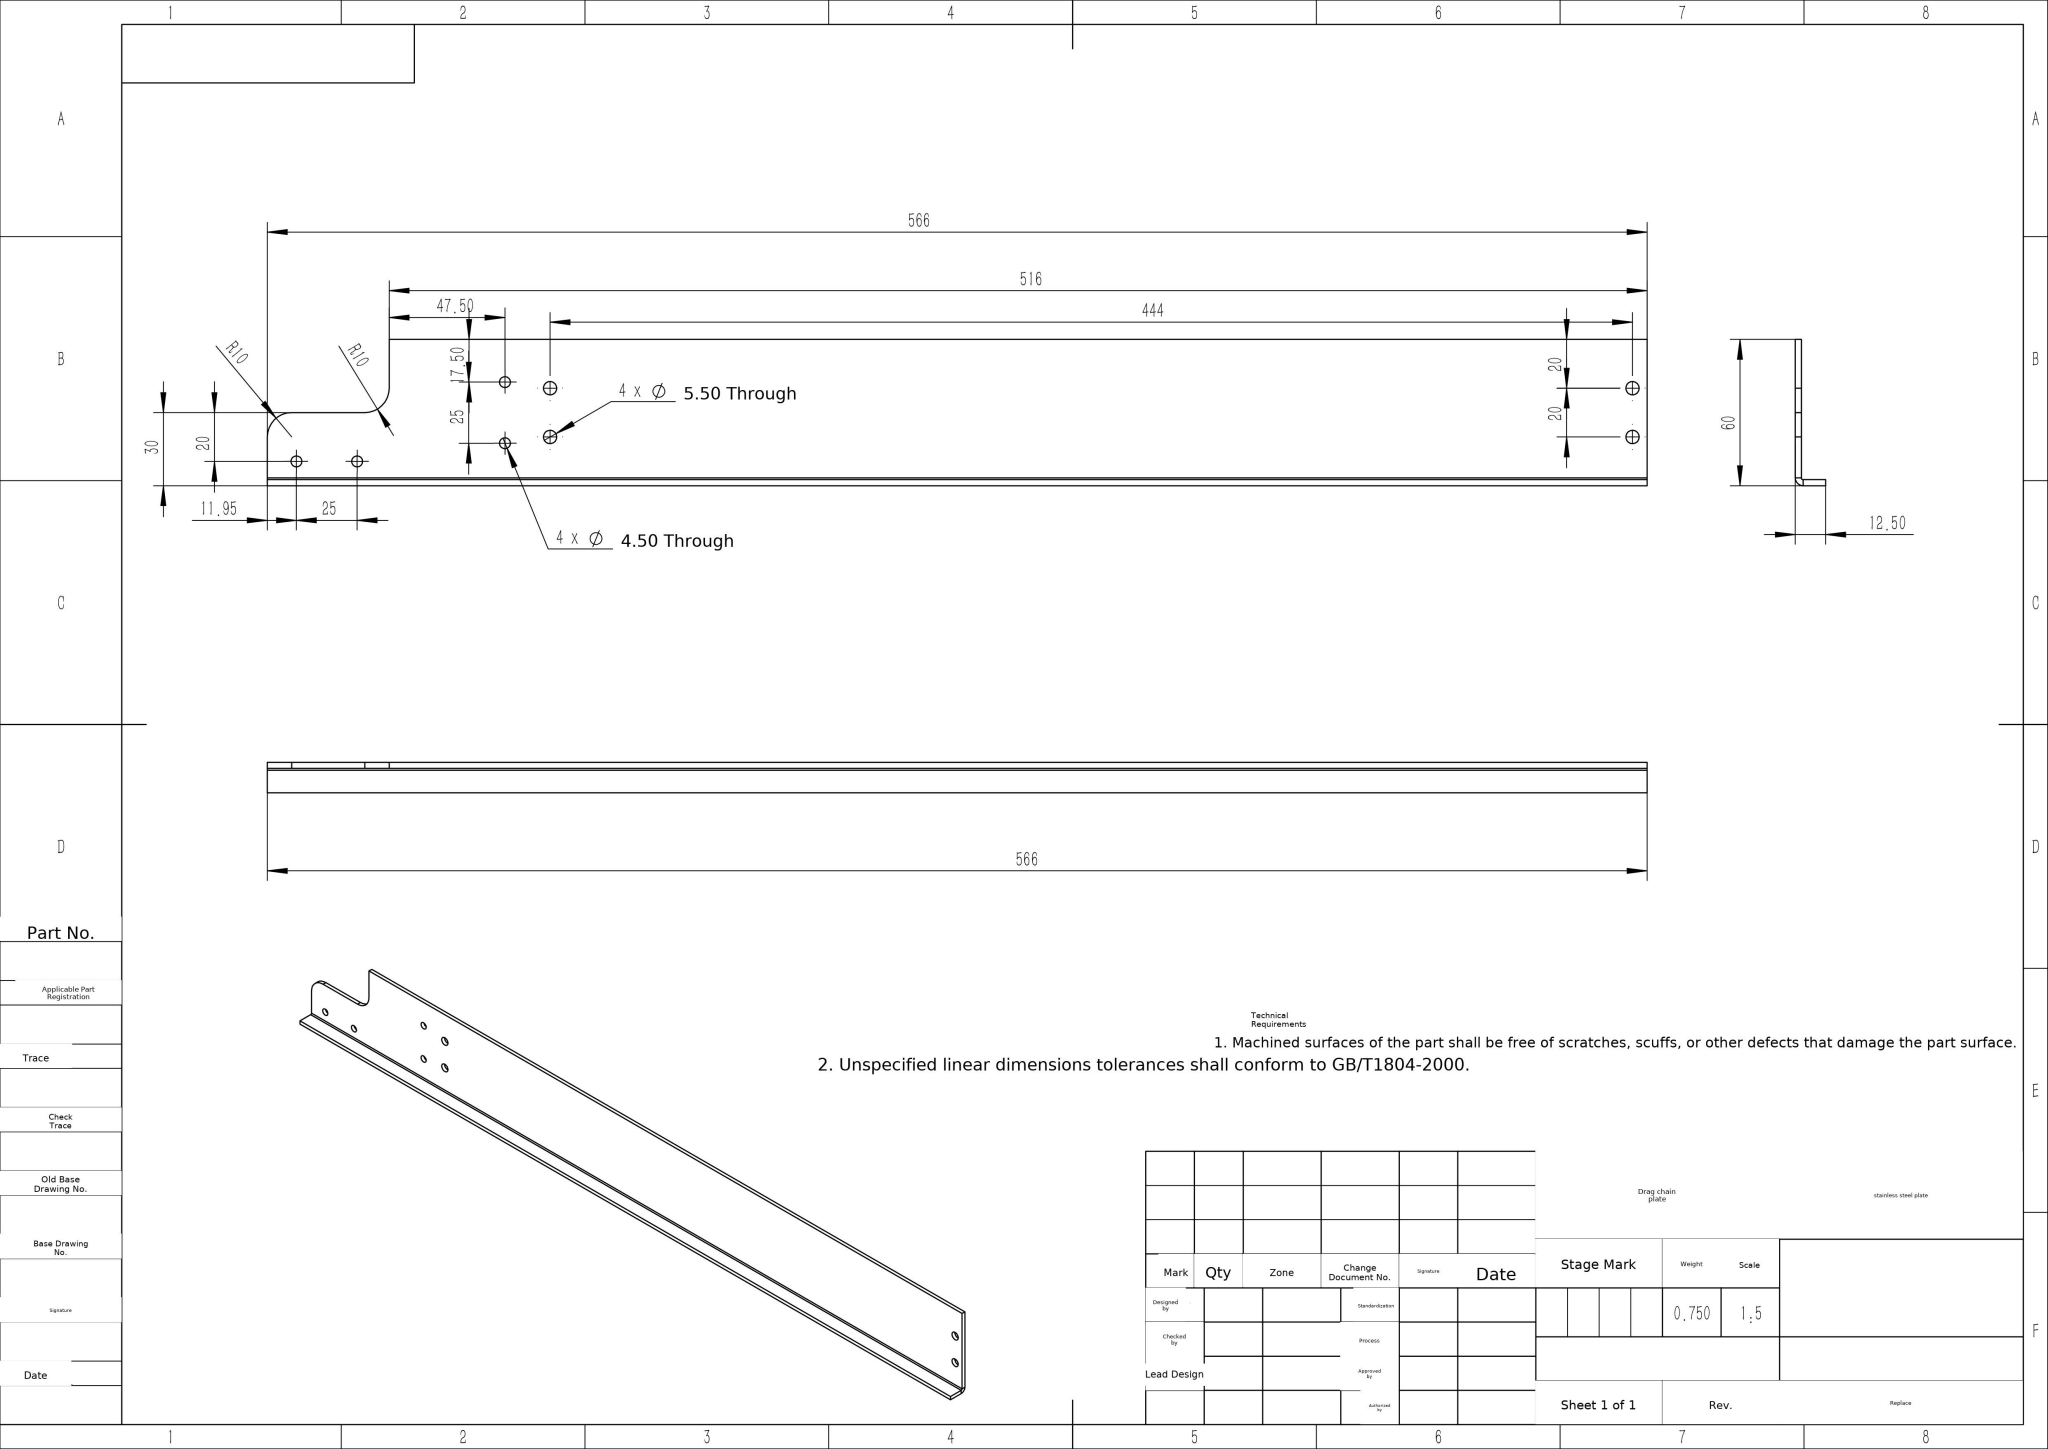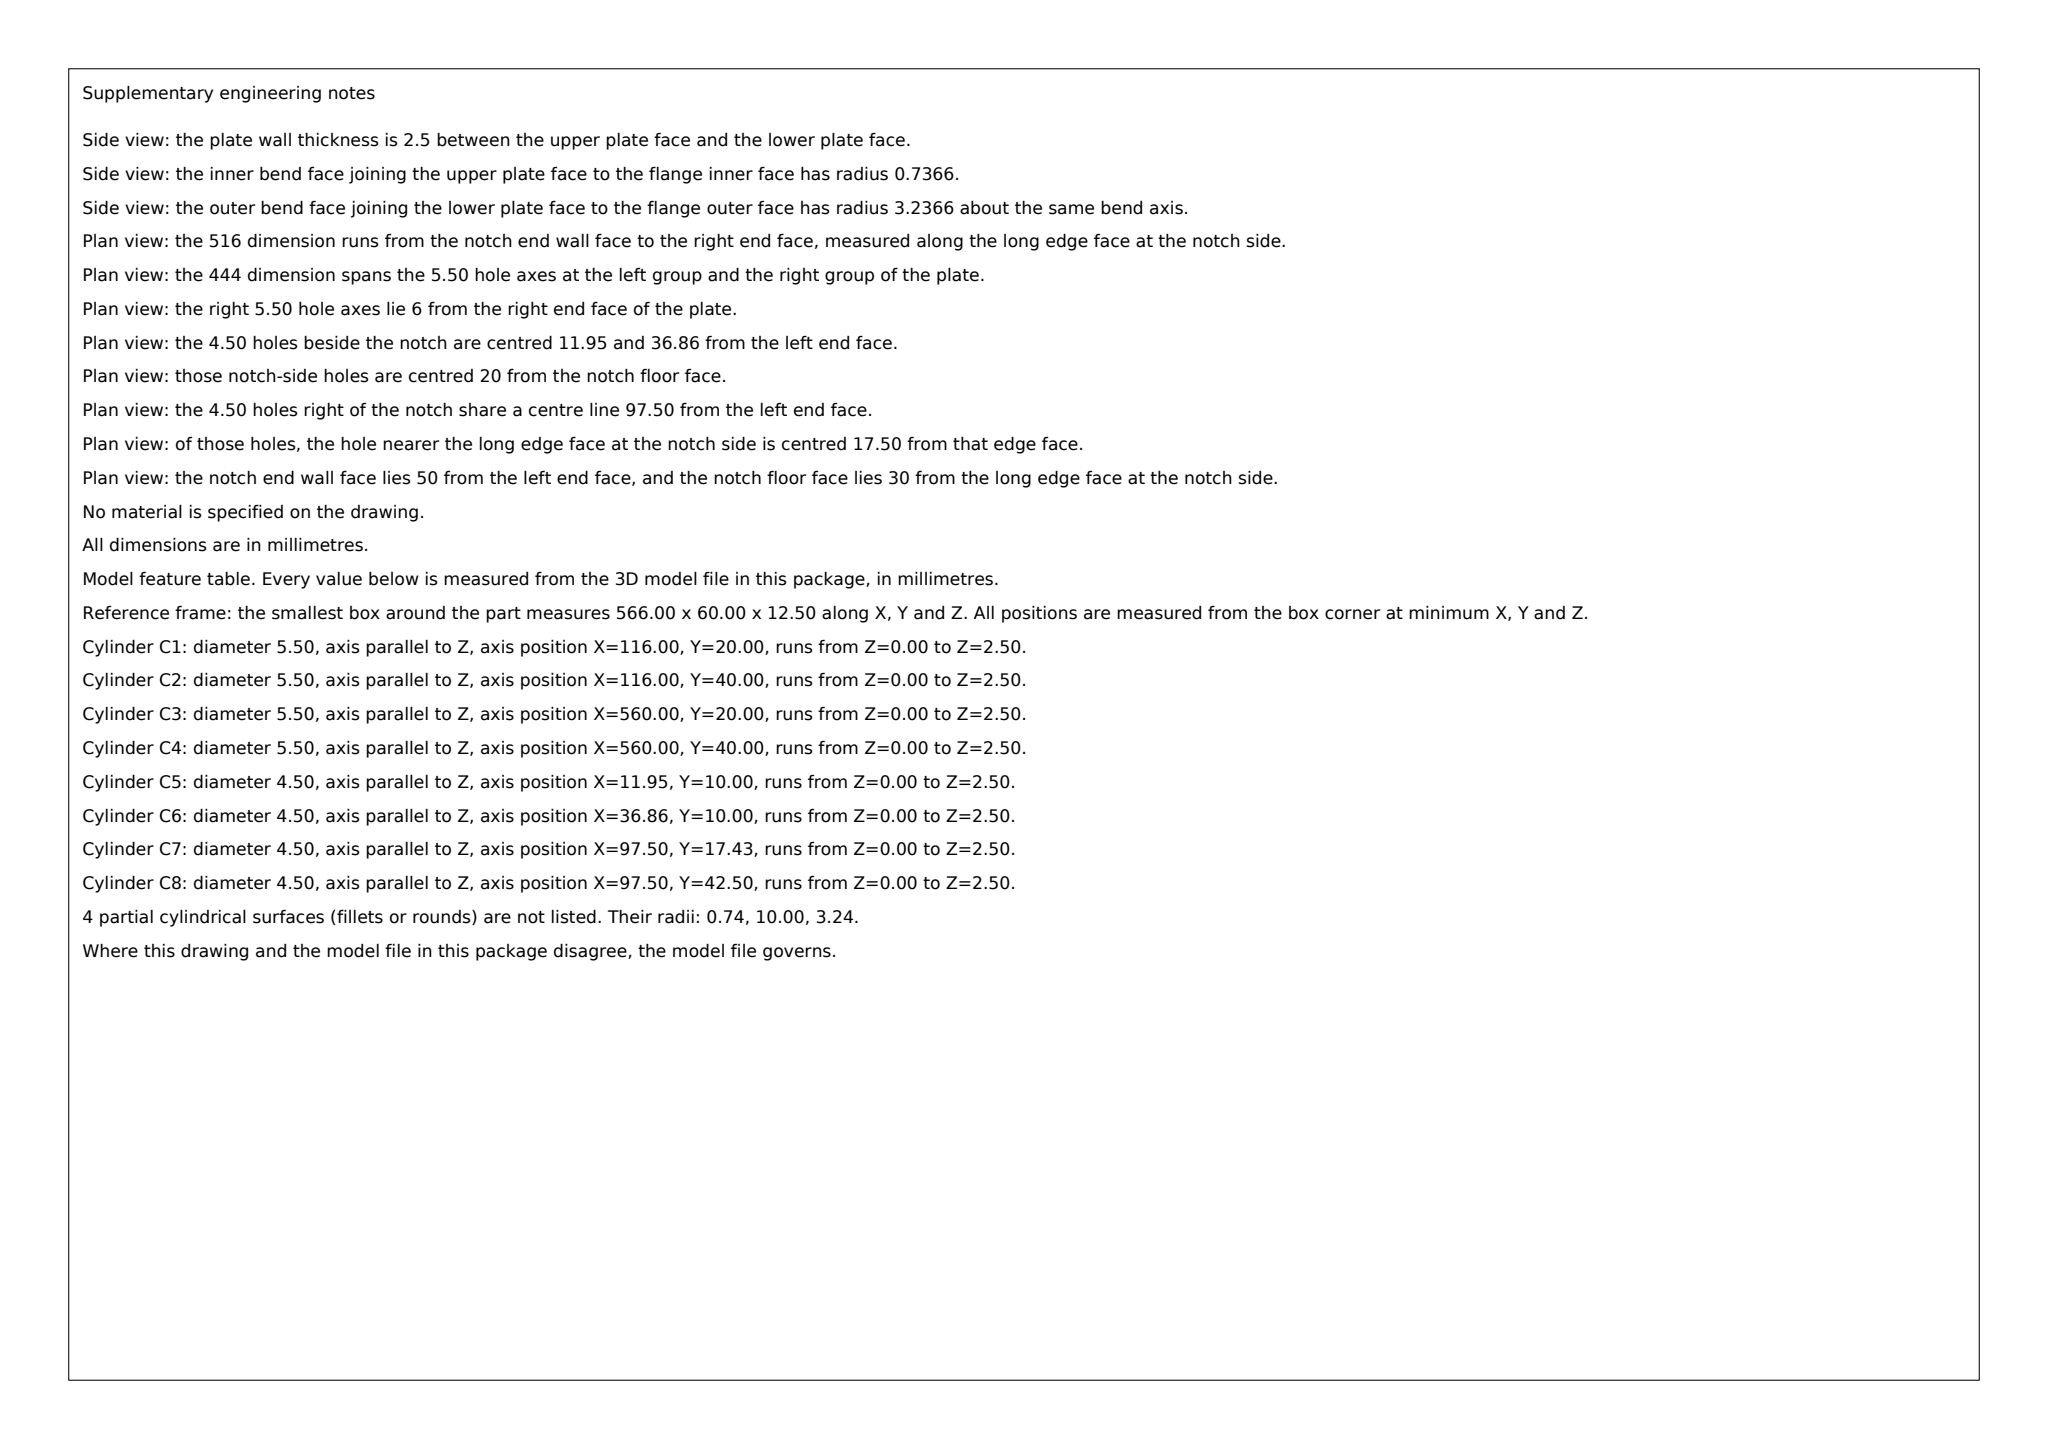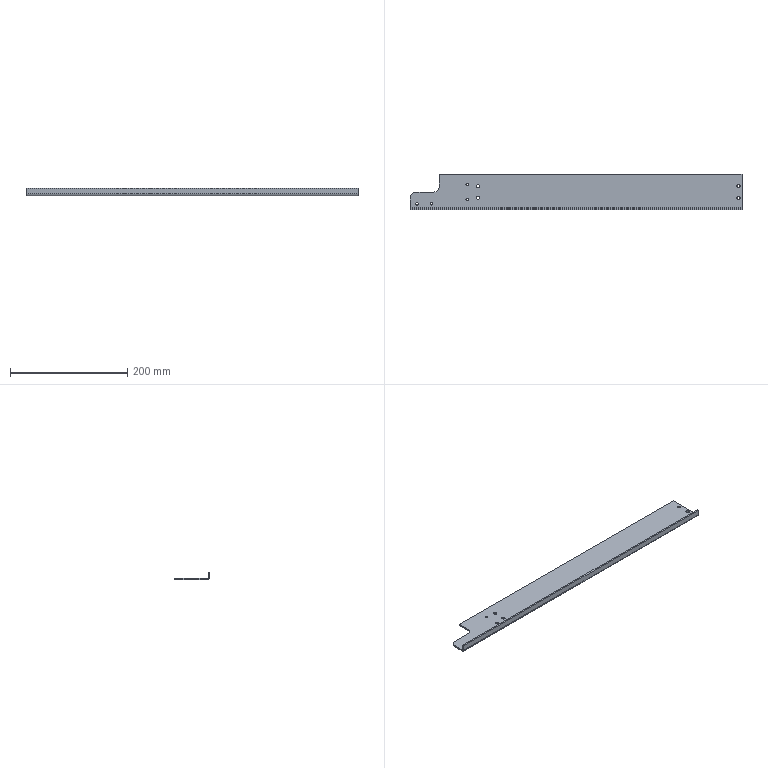Part | SolidWorks | mm | 1 solid | 34 faces | box 566 x 60 x 12.5 mm | volume 93697 mm3 | cylinder 20 | plane 14 | commonest cylinder face diameters 5.5 x8 4.5 x8 20 x2 6.473 x1 1.473 x1
Drawing notes:
BASE PLATE WIDTH 60 OVERALL FROM BENT WALL OUTER FACE | from the solid: bbox_xyz y=60.0; y planes at 0.0 (wall outer face) and 60.0 (top edge)
2X Ø4.50 AT LEFT: 10 FROM BENT WALL OUTER FACE (Y) | from the solid: cylinders dia 4.5 at [11.95,10.0] and [36.86,10.0], axis z
4X Ø5.50 GROUP: 116 FROM LEFT END, 6 FROM RIGHT END | from the solid: dia 5.5 holes at x=116.0 and x=560.0; bbox x=566.0 (566-560=6, spacing 444)
NOTCH AT LEFT END: 50 LG x 30 DP FROM TOP EDGE | from the solid: x plane at 50.0; y plane at 30.0 with bbox y=60.0 (566-516=50)